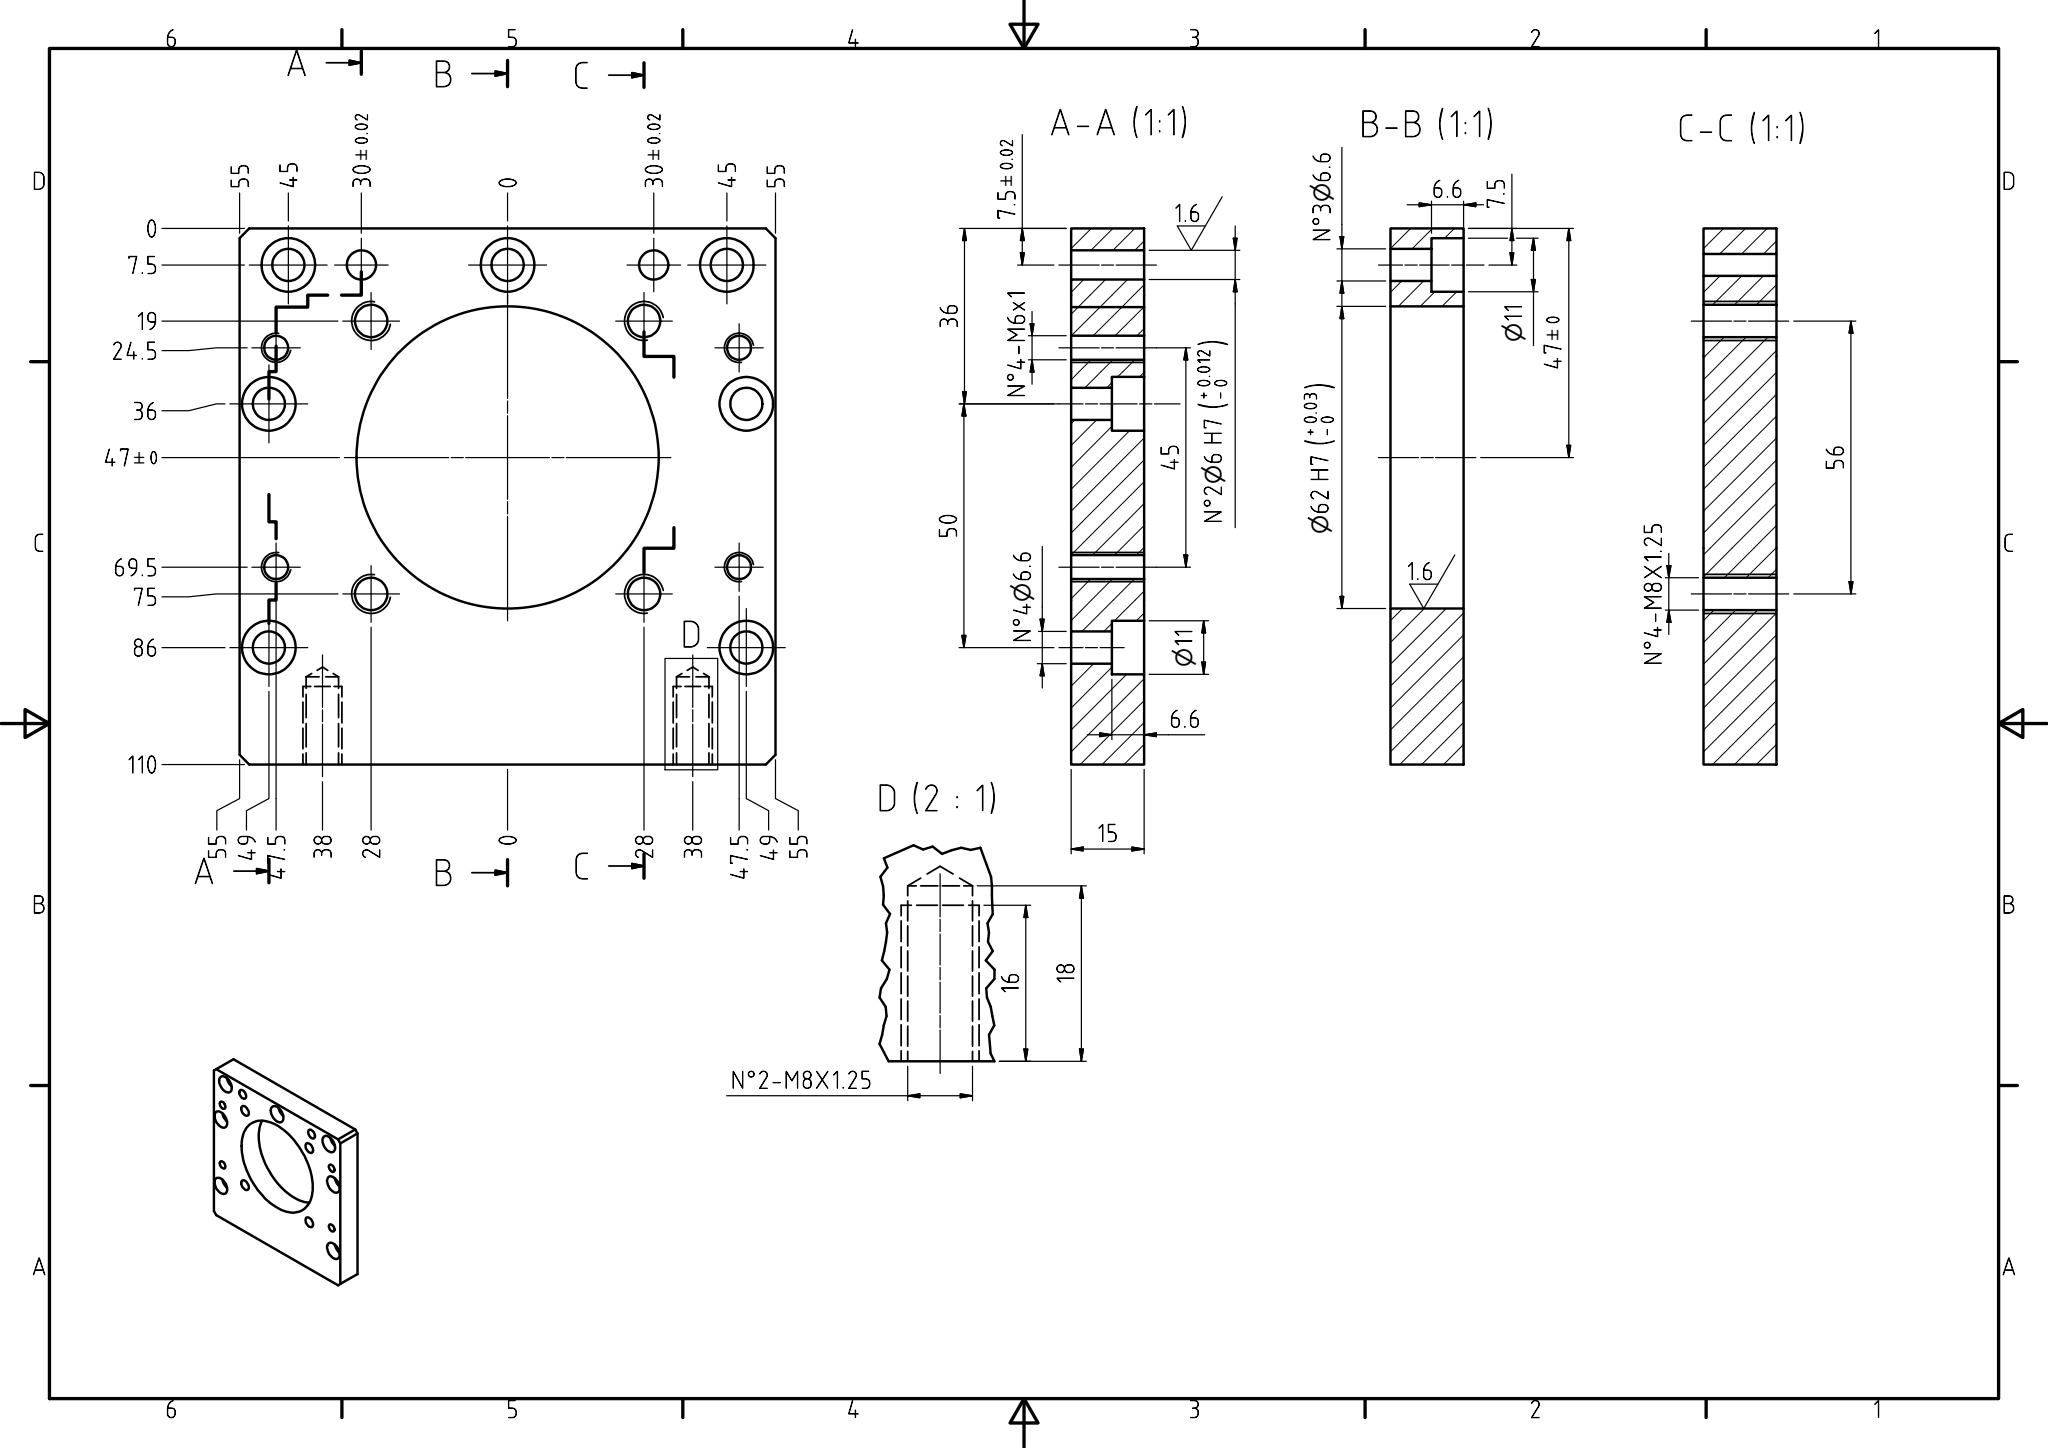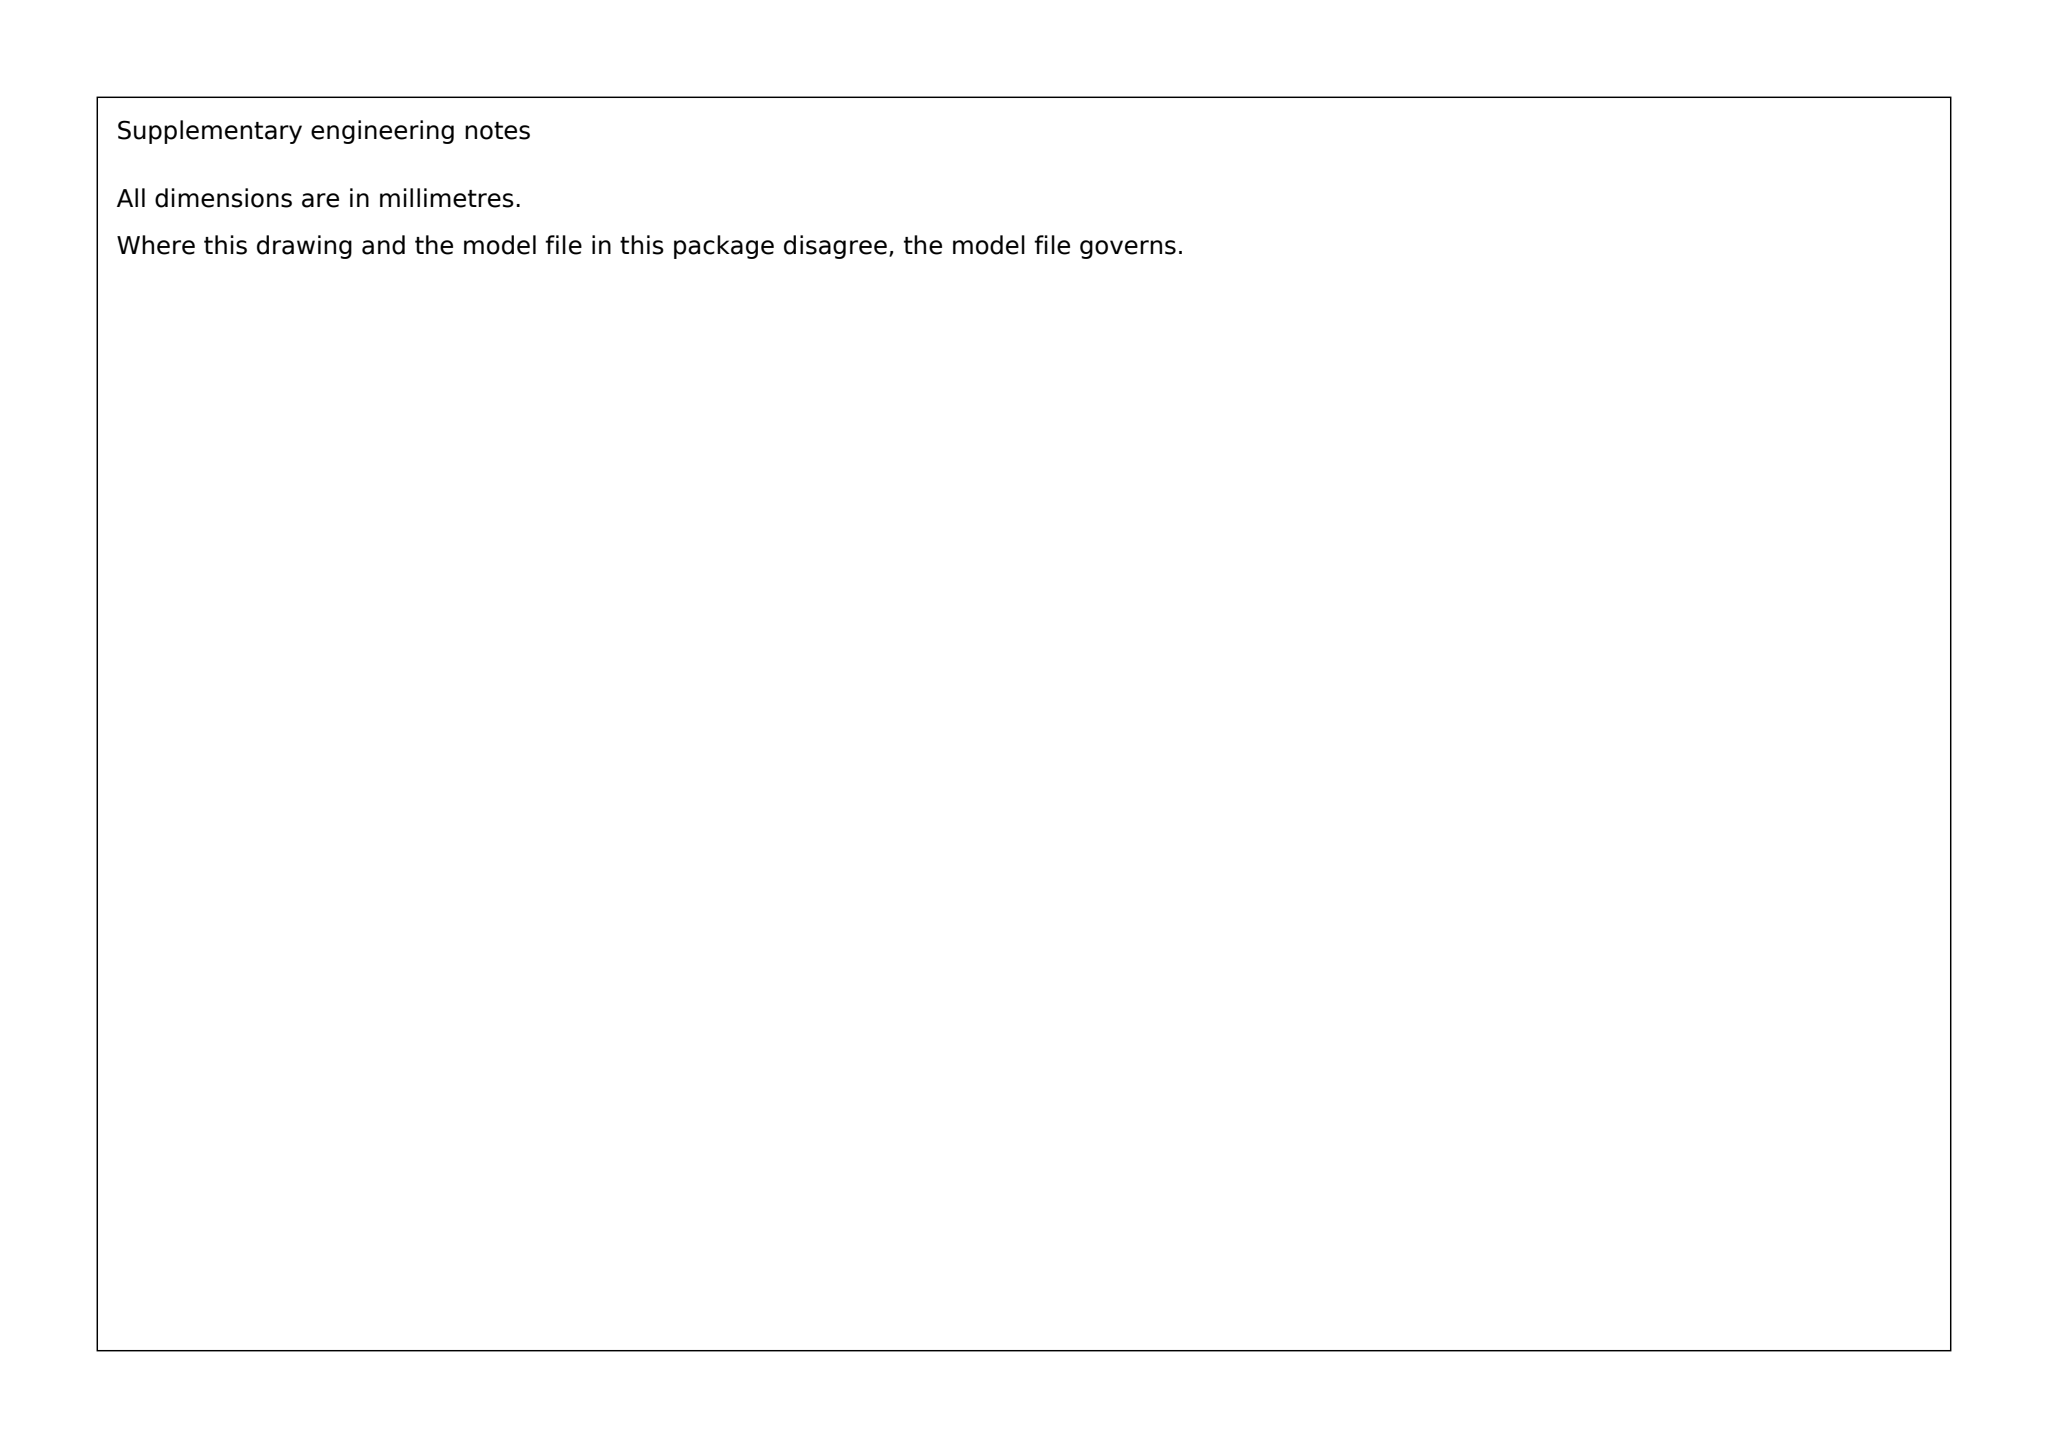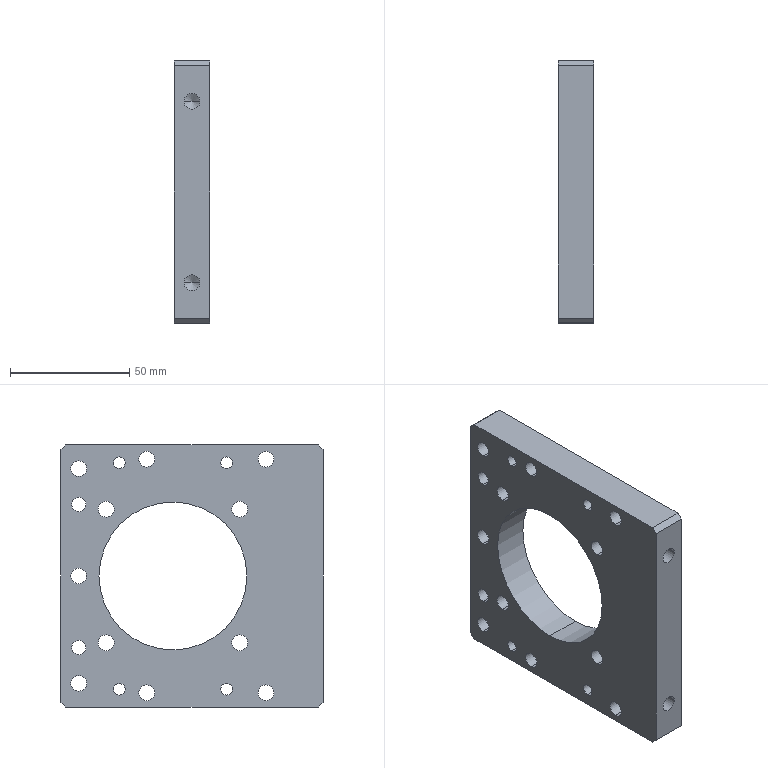Part | SolidWorks | mm | 1 solid | 75 faces | box 15 x 110 x 110 mm | volume 124327 mm3 | cylinder 54 | plane 17 | cone 4 | commonest cylinder face diameters 6.6 x14 11 x14 6.647 x12 4.917 x8 6 x4 62 x2